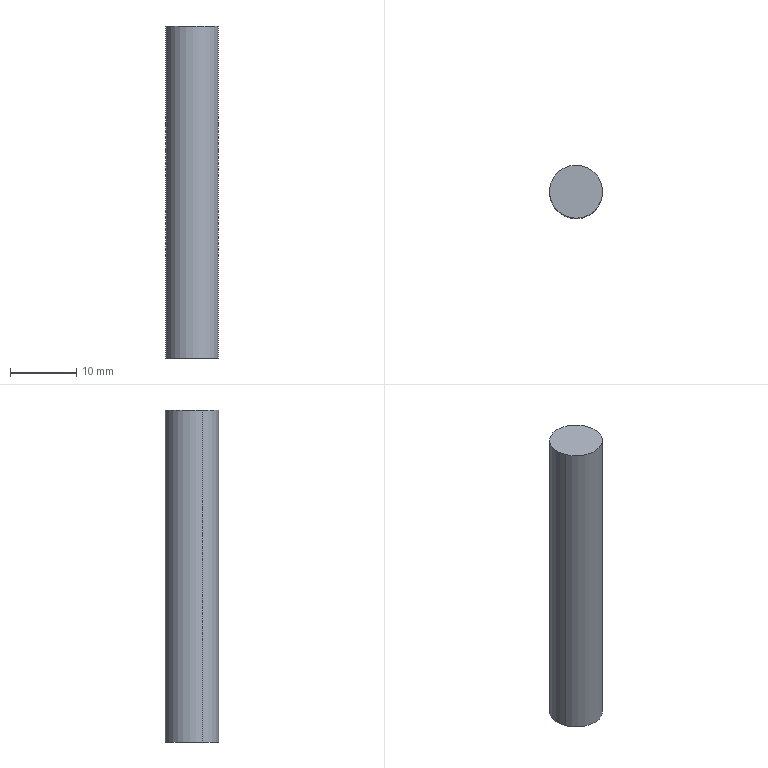Component | SolidWorks | Axis-1 | 1 solid | 4 faces | box 8 x 8 x 50 mm | volume 2513 mm3 | cylinder 2 | plane 2 | commonest cylinder face diameters 8 x2
build123d program:
from build123d import *

# Parameters (mm, degrees)
SKETCH1_R           = 4
BOSS_EXTRUDE1_DEPTH = 50


with BuildPart() as part:
    # Sketch1 → Boss-Extrude1 (new body)
    with BuildSketch(Plane.XY):
        Circle(SKETCH1_R)
    extrude(amount=BOSS_EXTRUDE1_DEPTH)


solid = part.part

# Placed as in the assembly
solid = solid.moved(Location((6.125, -1.646, -2.5), (0, 0, 0)))
STEP:
#1=COLOUR_RGB('',0.7922,0.8196,0.9333);
#2=FILL_AREA_STYLE_COLOUR('',#1);
#3=FILL_AREA_STYLE('',(#2));
#4=SURFACE_STYLE_FILL_AREA(#3);
#5=SURFACE_SIDE_STYLE('',(#4));
#6=SURFACE_STYLE_USAGE(.BOTH.,#5);
#7=PRESENTATION_STYLE_ASSIGNMENT((#6));
#8=CARTESIAN_POINT('',(0.3866,-0.004499,-0.09843));
#9=VERTEX_POINT('',#8);
#10=CARTESIAN_POINT('',(0.09567,-0.1251,-0.09843));
#11=VERTEX_POINT('',#10);
#12=CARTESIAN_POINT('',(0.2411,-0.06482,-0.09843));
#13=DIRECTION('',(0.,0.,-1.));
#14=DIRECTION('',(0.9237,0.383,0.));
#15=AXIS2_PLACEMENT_3D('',#12,#13,#14);
#16=CIRCLE('',#15,0.1575);
#17=EDGE_CURVE('',#9,#11,#16,.T.);
#18=ORIENTED_EDGE('',*,*,#17,.F.);
#19=CARTESIAN_POINT('',(0.3866,-0.004499,1.87));
#20=VERTEX_POINT('',#19);
#21=CARTESIAN_POINT('',(0.3866,-0.004499,-0.09843));
#22=DIRECTION('',(0.,0.,1.));
#23=VECTOR('',#22,39.37);
#24=LINE('',#21,#23);
#25=EDGE_CURVE('',#9,#20,#24,.T.);
#26=ORIENTED_EDGE('',*,*,#25,.T.);
#27=CARTESIAN_POINT('',(0.09567,-0.1251,1.87));
#28=VERTEX_POINT('',#27);
#29=CARTESIAN_POINT('',(0.2411,-0.06482,1.87));
#30=DIRECTION('',(0.,0.,-1.));
#31=DIRECTION('',(0.9237,0.383,0.));
#32=AXIS2_PLACEMENT_3D('',#29,#30,#31);
#33=CIRCLE('',#32,0.1575);
#34=EDGE_CURVE('',#20,#28,#33,.T.);
#35=ORIENTED_EDGE('',*,*,#34,.T.);
#36=CARTESIAN_POINT('',(0.09567,-0.1251,-0.09843));
#37=DIRECTION('',(0.,0.,1.));
#38=VECTOR('',#37,39.37);
#39=LINE('',#36,#38);
#40=EDGE_CURVE('',#11,#28,#39,.T.);
#41=ORIENTED_EDGE('',*,*,#40,.F.);
#42=EDGE_LOOP('',(#18,#26,#35,#41));
#43=FACE_OUTER_BOUND('',#42,.T.);
#44=CARTESIAN_POINT('',(0.2411,-0.06482,-0.09843));
#45=DIRECTION('',(0.,0.,1.));
#46=DIRECTION('',(-0.9237,-0.383,0.));
#47=AXIS2_PLACEMENT_3D('',#44,#45,#46);
#48=CYLINDRICAL_SURFACE('',#47,0.1575);
#49=ADVANCED_FACE('',(#43),#48,.T.);
#50=ORIENTED_EDGE('',*,*,#25,.F.);
#51=CARTESIAN_POINT('',(0.2411,-0.06482,-0.09843));
#52=DIRECTION('',(0.,0.,-1.));
#53=DIRECTION('',(0.9237,0.383,0.));
#54=AXIS2_PLACEMENT_3D('',#51,#52,#53);
#55=CIRCLE('',#54,0.1575);
#56=EDGE_CURVE('',#11,#9,#55,.T.);
#57=ORIENTED_EDGE('',*,*,#56,.F.);
#58=ORIENTED_EDGE('',*,*,#40,.T.);
#59=CARTESIAN_POINT('',(0.2411,-0.06482,1.87));
#60=DIRECTION('',(0.,0.,-1.));
#61=DIRECTION('',(0.9237,0.383,0.));
#62=AXIS2_PLACEMENT_3D('',#59,#60,#61);
#63=CIRCLE('',#62,0.1575);
#64=EDGE_CURVE('',#28,#20,#63,.T.);
#65=ORIENTED_EDGE('',*,*,#64,.T.);
#66=EDGE_LOOP('',(#50,#57,#58,#65));
#67=FACE_OUTER_BOUND('',#66,.T.);
#68=CARTESIAN_POINT('',(0.2411,-0.06482,-0.09843));
#69=DIRECTION('',(0.,0.,1.));
#70=DIRECTION('',(-0.9237,-0.383,0.));
#71=AXIS2_PLACEMENT_3D('',#68,#69,#70);
#72=CYLINDRICAL_SURFACE('',#71,0.1575);
#73=ADVANCED_FACE('',(#67),#72,.T.);
#74=ORIENTED_EDGE('',*,*,#56,.T.);
#75=ORIENTED_EDGE('',*,*,#17,.T.);
#76=EDGE_LOOP('',(#74,#75));
#77=FACE_OUTER_BOUND('',#76,.T.);
#78=CARTESIAN_POINT('',(0.2411,-0.06482,-0.09843));
#79=DIRECTION('',(0.,0.,-1.));
#80=DIRECTION('',(0.9237,0.383,0.));
#81=AXIS2_PLACEMENT_3D('',#78,#79,#80);
#82=PLANE('',#81);
#83=ADVANCED_FACE('',(#77),#82,.T.);
#84=ORIENTED_EDGE('',*,*,#64,.F.);
#85=ORIENTED_EDGE('',*,*,#34,.F.);
#86=EDGE_LOOP('',(#84,#85));
#87=FACE_OUTER_BOUND('',#86,.T.);
#88=CARTESIAN_POINT('',(0.2411,-0.06482,1.87));
#89=DIRECTION('',(0.,0.,-1.));
#90=DIRECTION('',(0.9237,0.383,0.));
#91=AXIS2_PLACEMENT_3D('',#88,#89,#90);
#92=PLANE('',#91);
#93=ADVANCED_FACE('',(#87),#92,.F.);
#94=CLOSED_SHELL('',(#49,#73,#83,#93));
#95=MANIFOLD_SOLID_BREP('',#94);
#96=STYLED_ITEM('',(#7),#95);
#97=PRESENTATION_LAYER_ASSIGNMENT('','',(#96));
#98=CARTESIAN_POINT('',(0.,0.,0.));
#99=DIRECTION('',(0.,0.,1.));
#100=DIRECTION('',(1.,0.,0.));
#101=AXIS2_PLACEMENT_3D('',#98,#99,#100);
#102=(LENGTH_UNIT()NAMED_UNIT(*)SI_UNIT($,.METRE.));
#103=LENGTH_MEASURE_WITH_UNIT(LENGTH_MEASURE(0.0254),#102);
#104=DIMENSIONAL_EXPONENTS(1.,0.,0.,0.,0.,0.,0.);
#105=(CONVERSION_BASED_UNIT('',#103)LENGTH_UNIT()NAMED_UNIT(#104));
#106=UNCERTAINTY_MEASURE_WITH_UNIT(LENGTH_MEASURE(0.00001),#105,'','');
#107=(NAMED_UNIT(*)PLANE_ANGLE_UNIT()SI_UNIT($,.RADIAN.));
#108=(NAMED_UNIT(*)SI_UNIT($,.STERADIAN.)SOLID_ANGLE_UNIT());
#109=(GEOMETRIC_REPRESENTATION_CONTEXT(3)GLOBAL_UNCERTAINTY_ASSIGNED_CONTEXT((#106))GLOBAL_UNIT_ASSIGNED_CONTEXT((#105,#107,#108))REPRESENTATION_CONTEXT('',''));
#110=ADVANCED_BREP_SHAPE_REPRESENTATION('',(#95,#101),#109);
#111=(LENGTH_UNIT()NAMED_UNIT(*)SI_UNIT($,.METRE.));
#112=LENGTH_MEASURE_WITH_UNIT(LENGTH_MEASURE(0.0254),#111);
#113=DIMENSIONAL_EXPONENTS(1.,0.,0.,0.,0.,0.,0.);
#114=(CONVERSION_BASED_UNIT('',#112)LENGTH_UNIT()NAMED_UNIT(#113));
#115=UNCERTAINTY_MEASURE_WITH_UNIT(LENGTH_MEASURE(0.00001),#114,'','');
#116=(NAMED_UNIT(*)PLANE_ANGLE_UNIT()SI_UNIT($,.RADIAN.));
#117=(NAMED_UNIT(*)SI_UNIT($,.STERADIAN.)SOLID_ANGLE_UNIT());
#118=(GEOMETRIC_REPRESENTATION_CONTEXT(3)GLOBAL_UNCERTAINTY_ASSIGNED_CONTEXT((#115))GLOBAL_UNIT_ASSIGNED_CONTEXT((#114,#116,#117))REPRESENTATION_CONTEXT('',''));
#119=MECHANICAL_DESIGN_GEOMETRIC_PRESENTATION_REPRESENTATION('',(#96),#118);